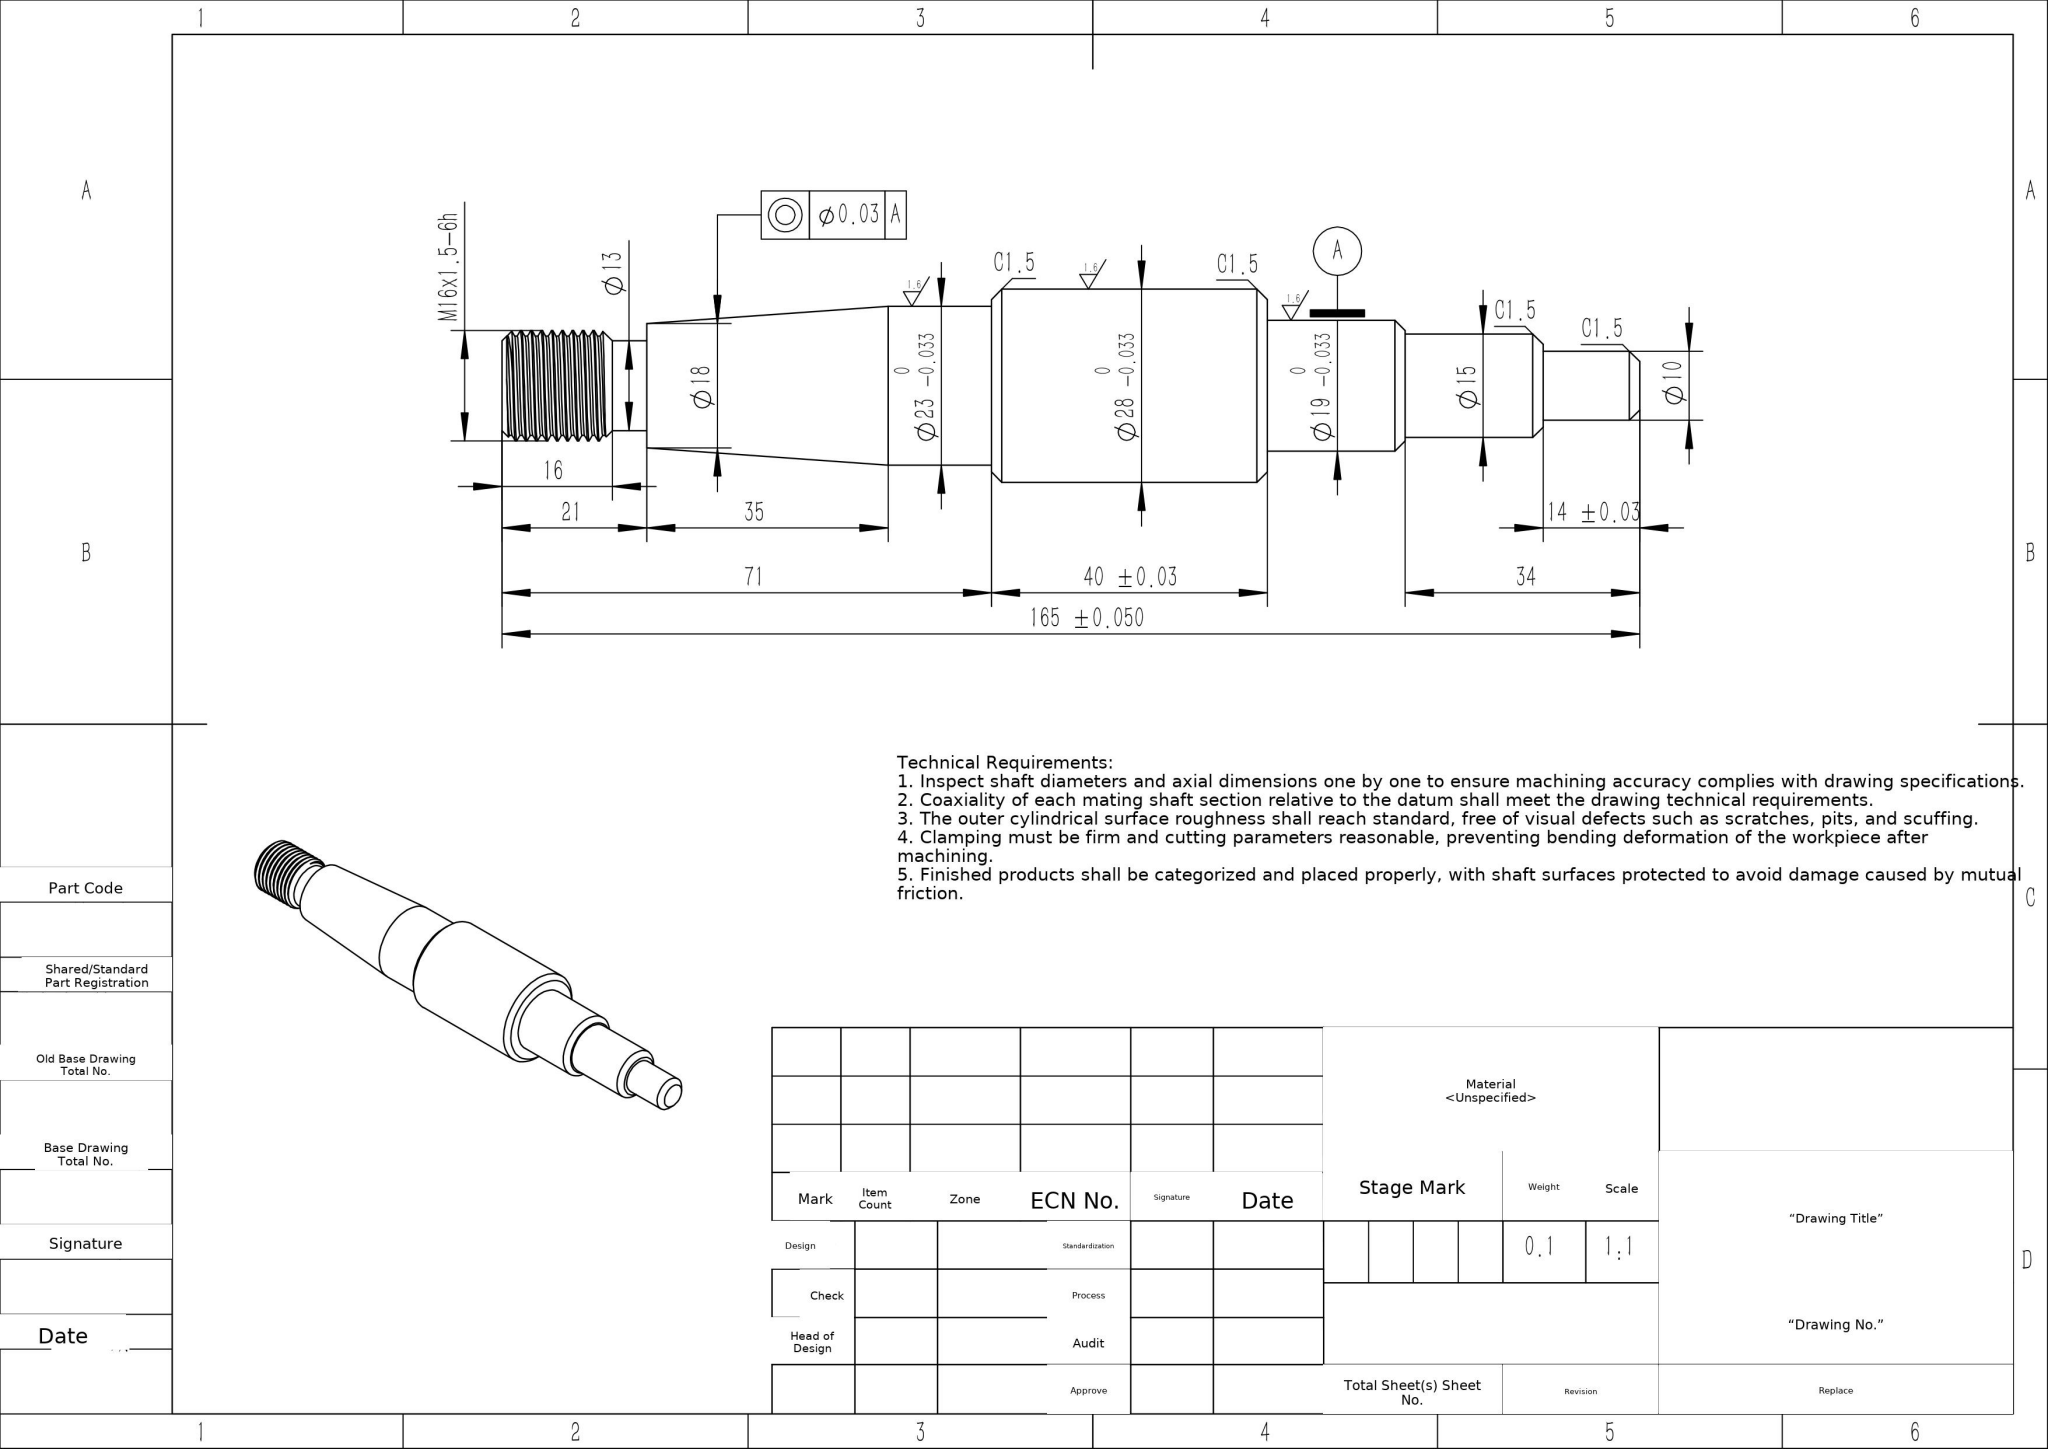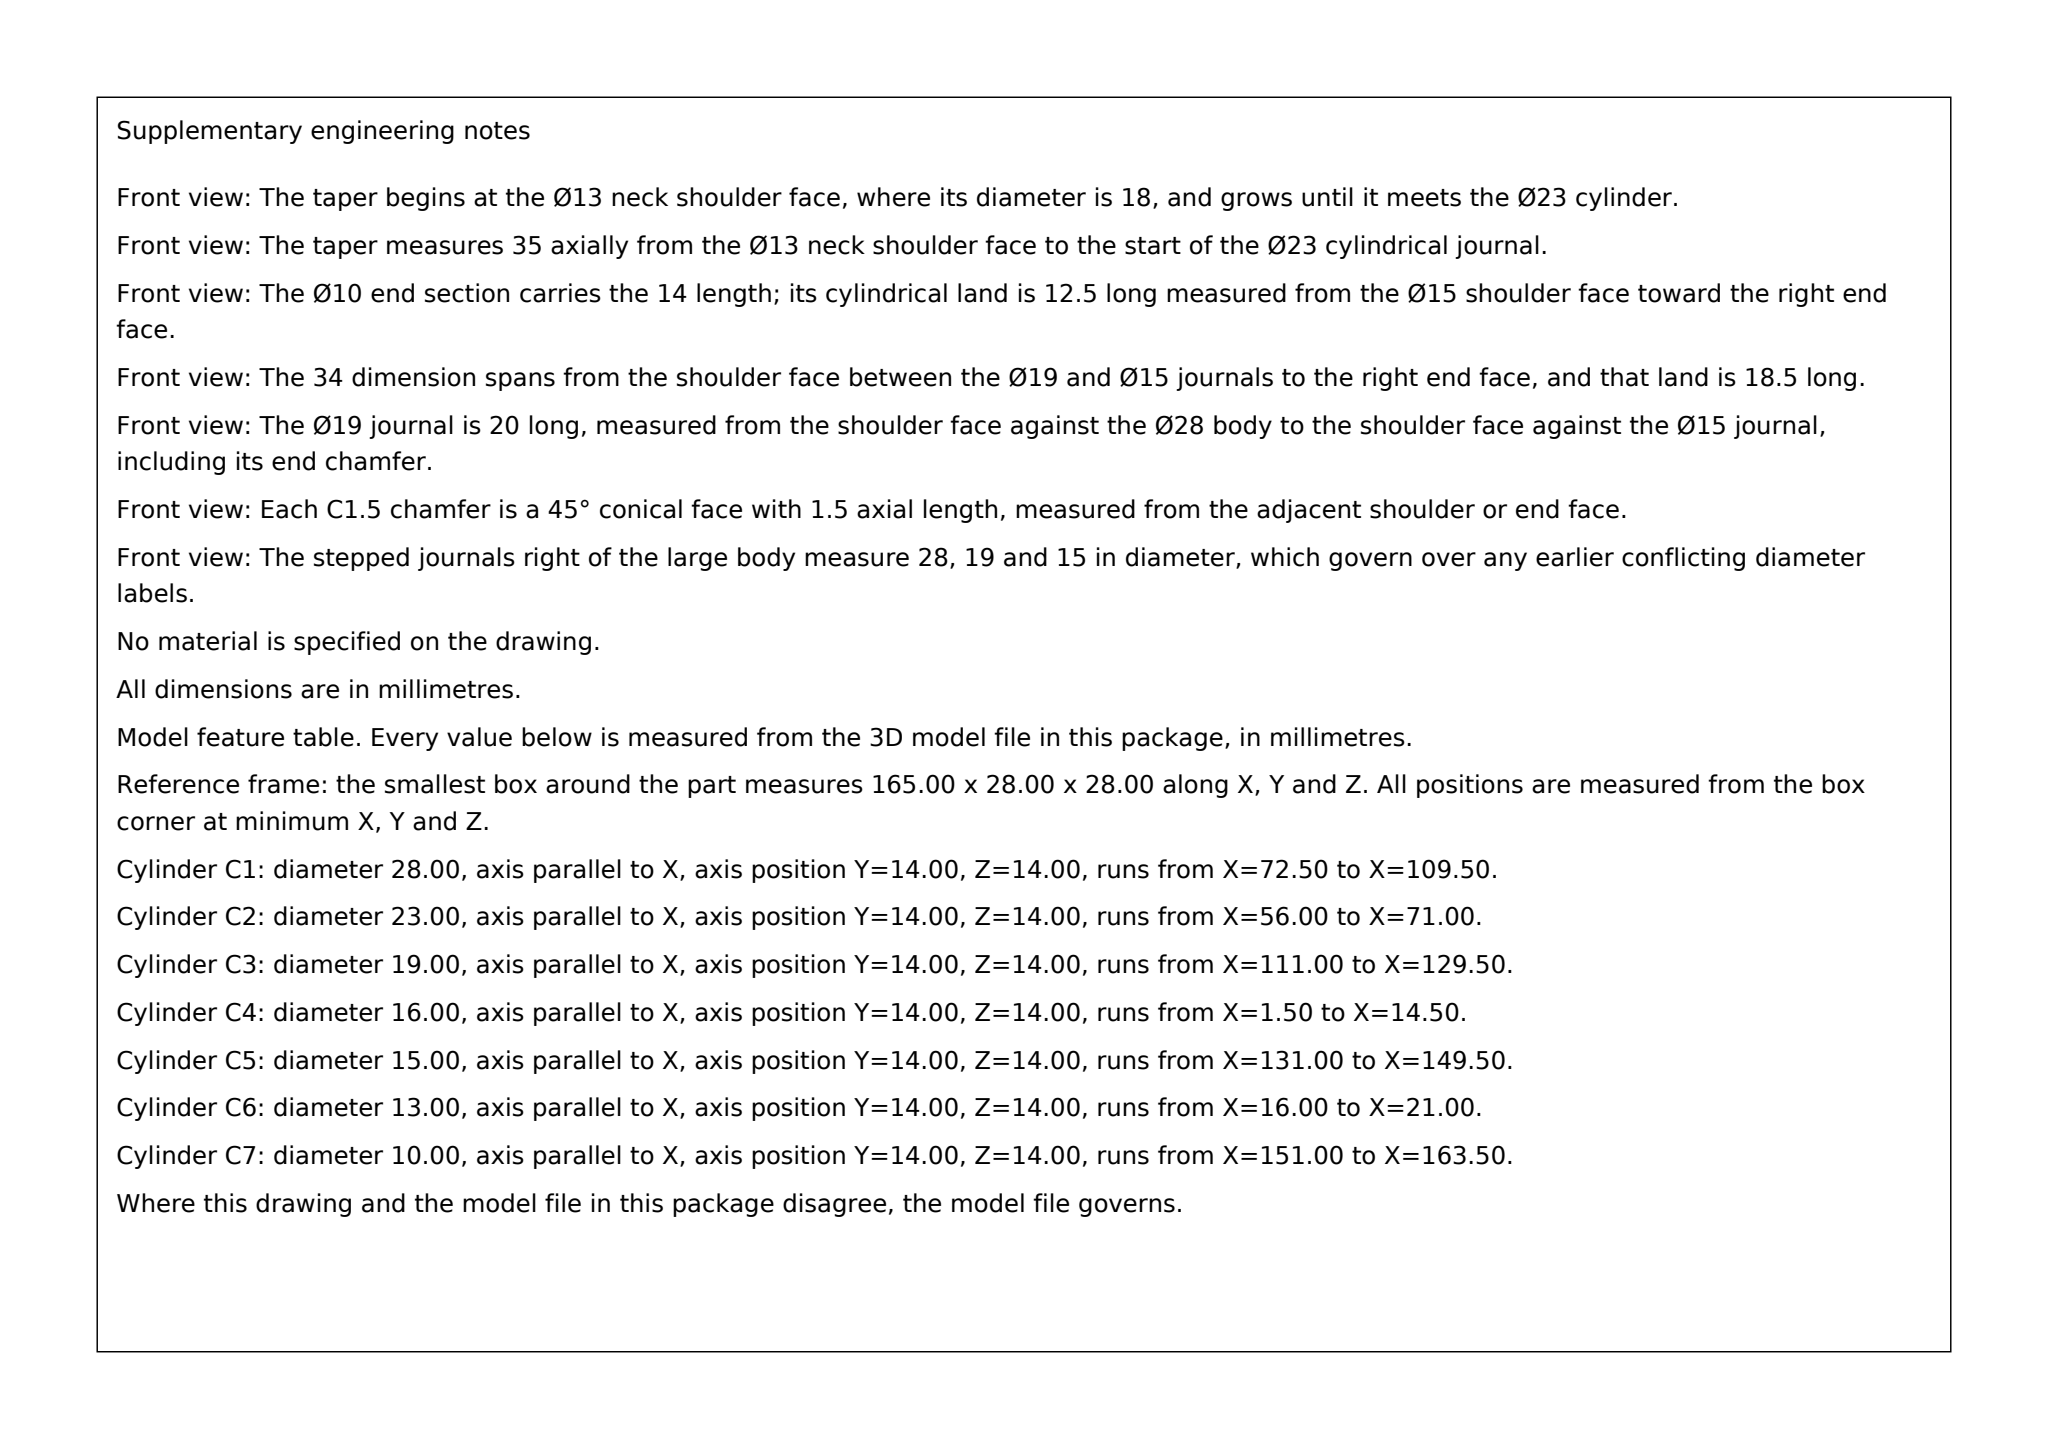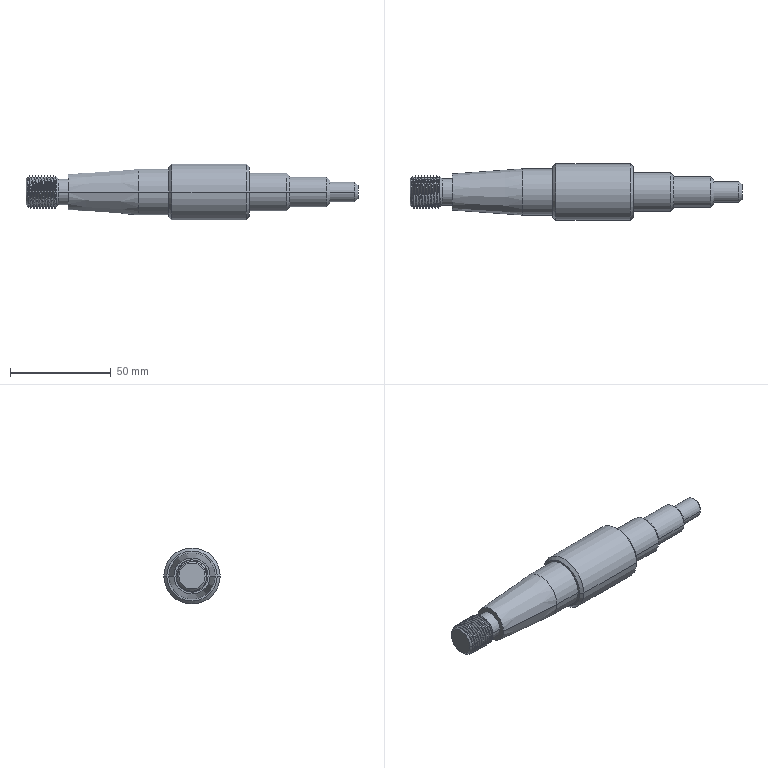Part | SolidWorks | mm | 1 solid | 57 faces | box 165 x 28 x 28 mm | volume 55908 mm3 | cylinder 30 | cone 17 | plane 7 | spline 3 | commonest cylinder face diameters 16 x18 10 x2 15 x2 19 x2 28 x2 23 x2 13 x2
Drawing notes:
CHAMFER AT Ø19/Ø15 STEP: C1.5 x 45°, 1 PL (NOT QTY 11) | from the solid: 90° cone at x=129.5, ref dia 16, axial size 1.5 between Ø19 shaft (111.0-129.5) and Ø15 shaft (131.0-149.5)
C1.4 x 45° AT FREE (LH) END OF M16x1.5-6h THD | from the solid: cone 90 deg, ref dia 16, bbox_from x=0.0, x-extent 1.4 (to x=1.4)
C1.5 x 45° AT THD RUN-OUT TO Ø13, FROM 14.5 TO 16 | from the solid: cone 90 deg, ref dia 13, bbox_from x=14.5, x-extent 1.5; Ø13 cyl x=16 to 21
M16x1.5-6h FULL THD 16 LG FROM LH END; Ø13 x 5 LG TO 21 | from the solid: thread crest arcs x=1.5-14.5, chamfers 0-1.4 & 14.5-16; Ø13 boss x=16-21; face plane x=21